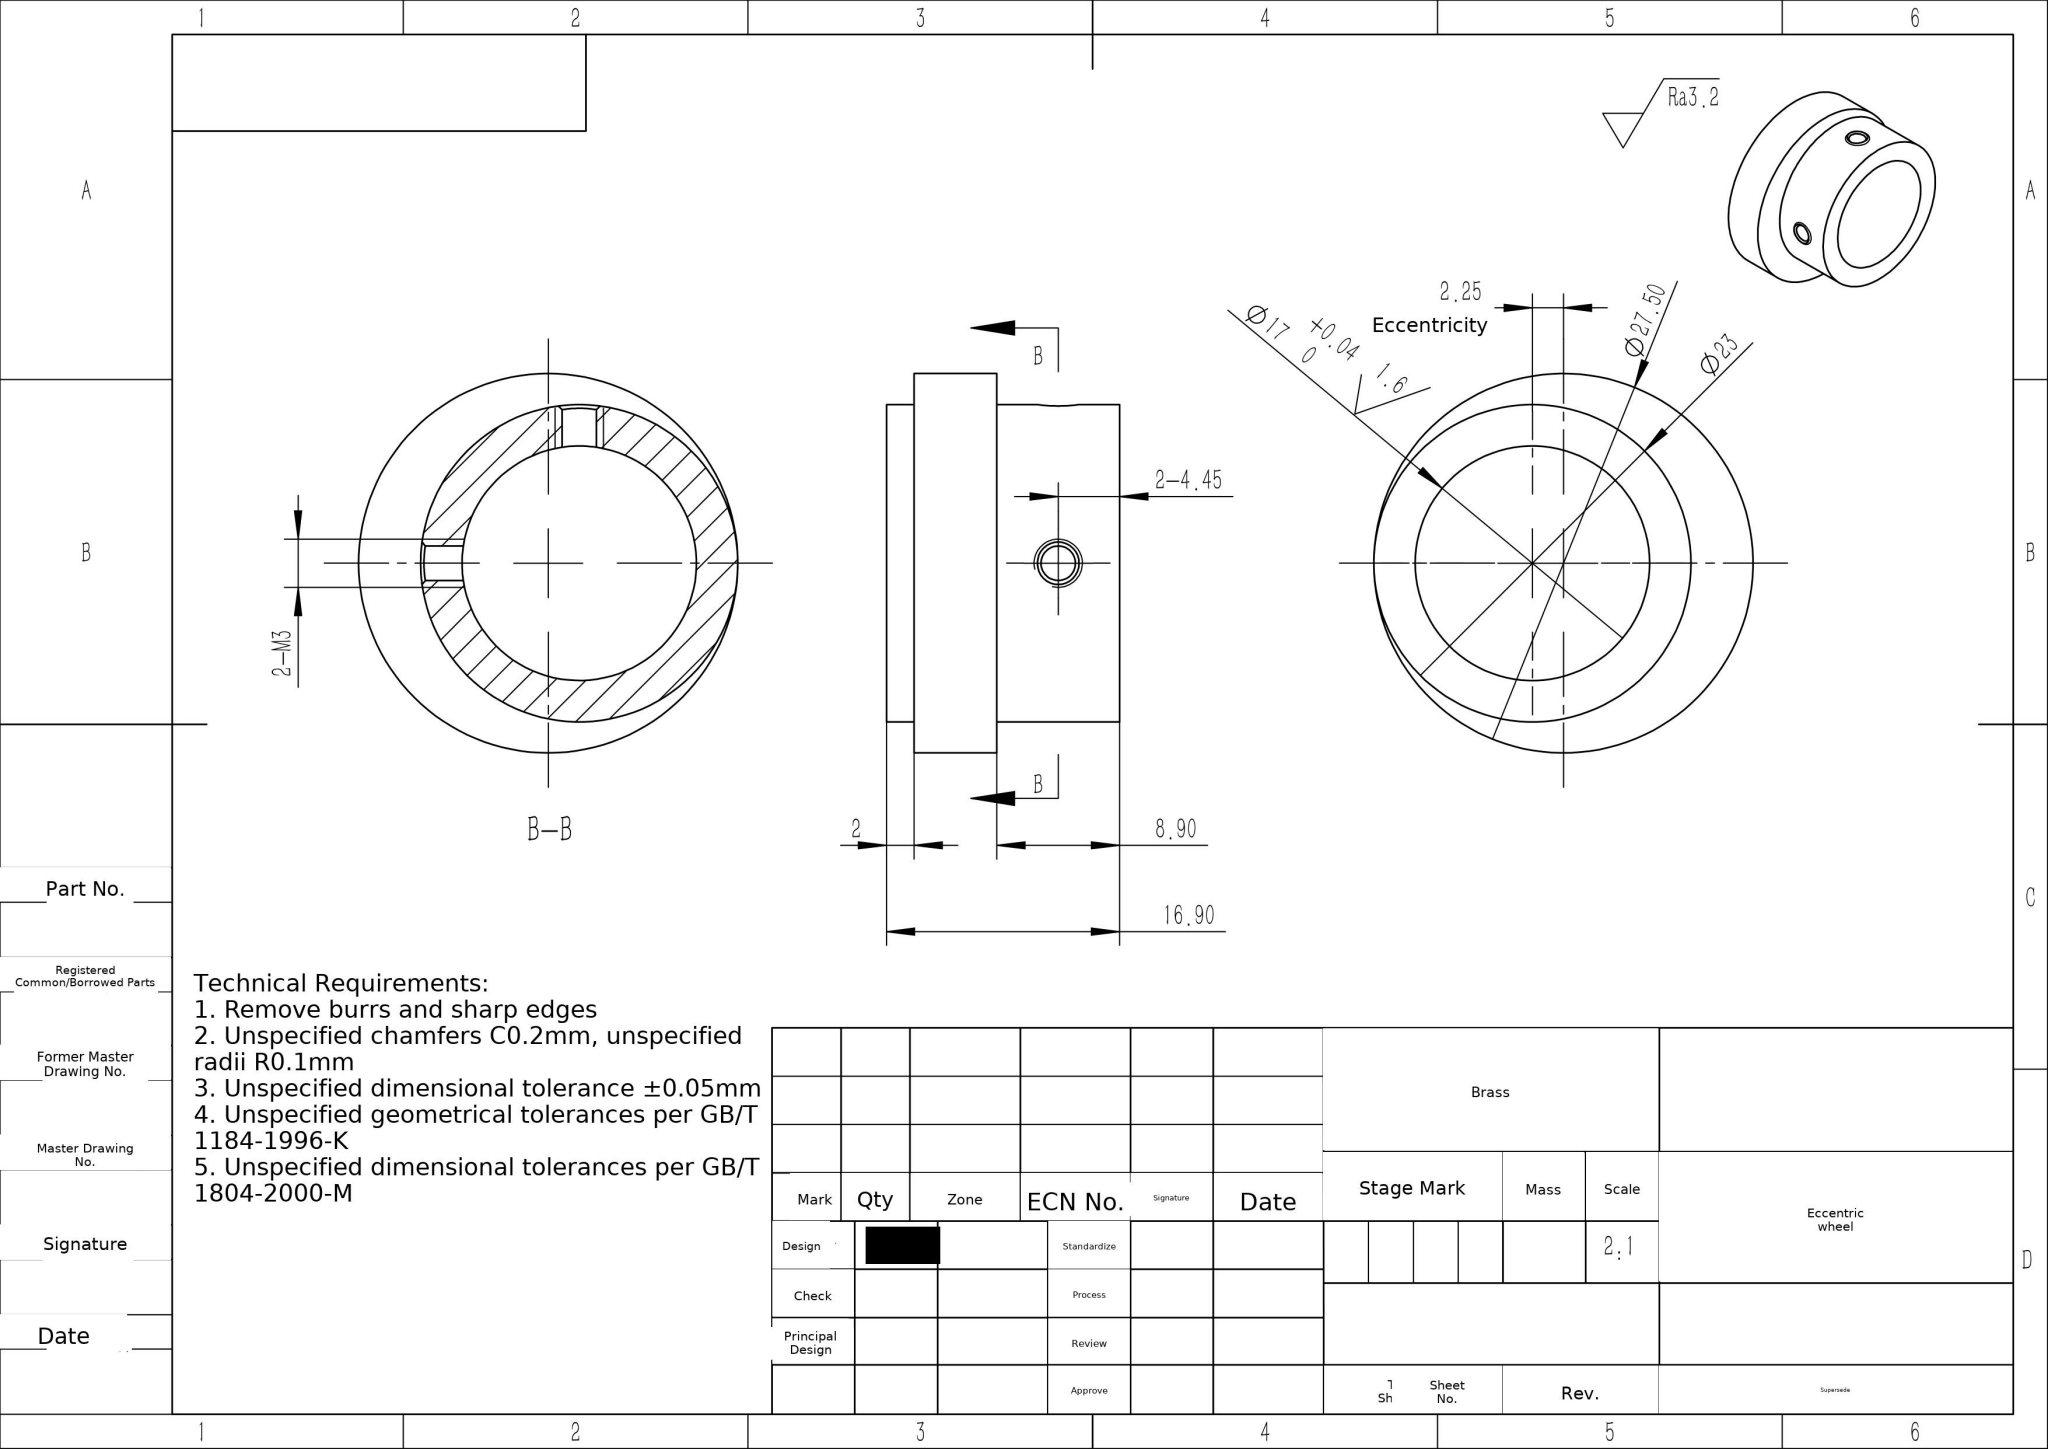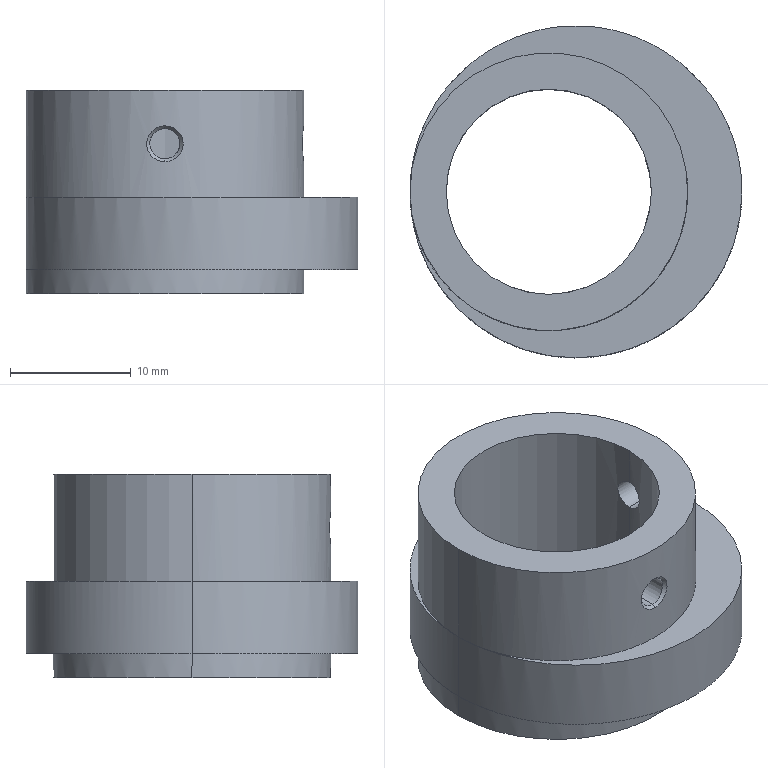Part | SolidWorks | mm | material Brass | 1 solid | 20 faces | box 27.5 x 27.5 x 16.9 mm | volume 4226 mm3 | cylinder 12 | spline 4 | plane 4 | commonest cylinder face diameters 2.5 x4 23 x4 27.5 x2 17 x2